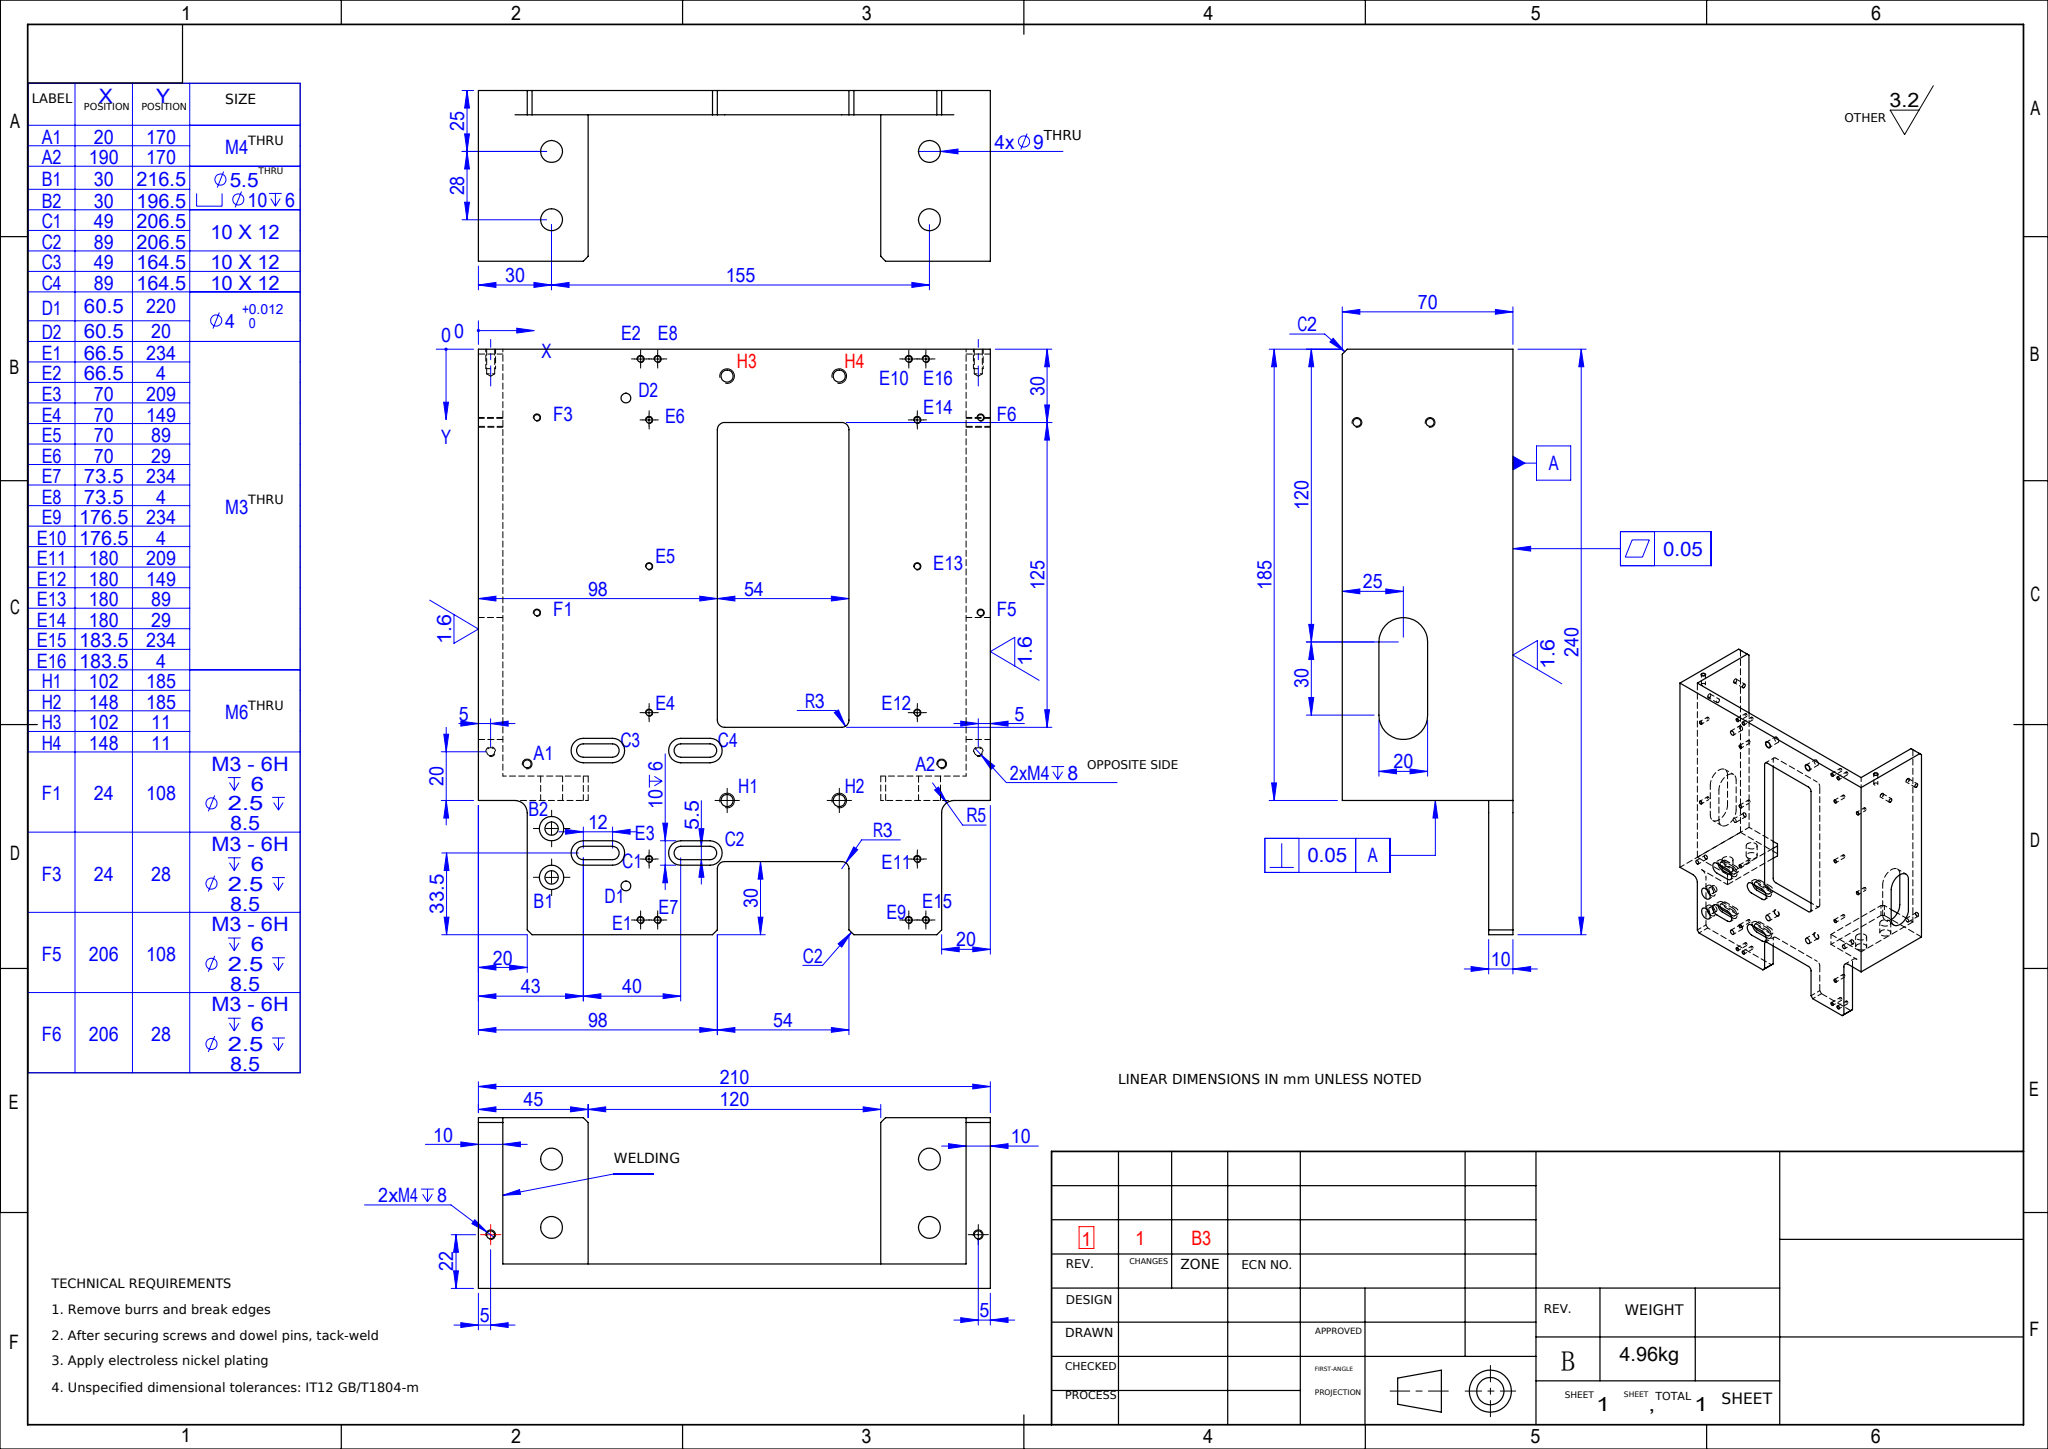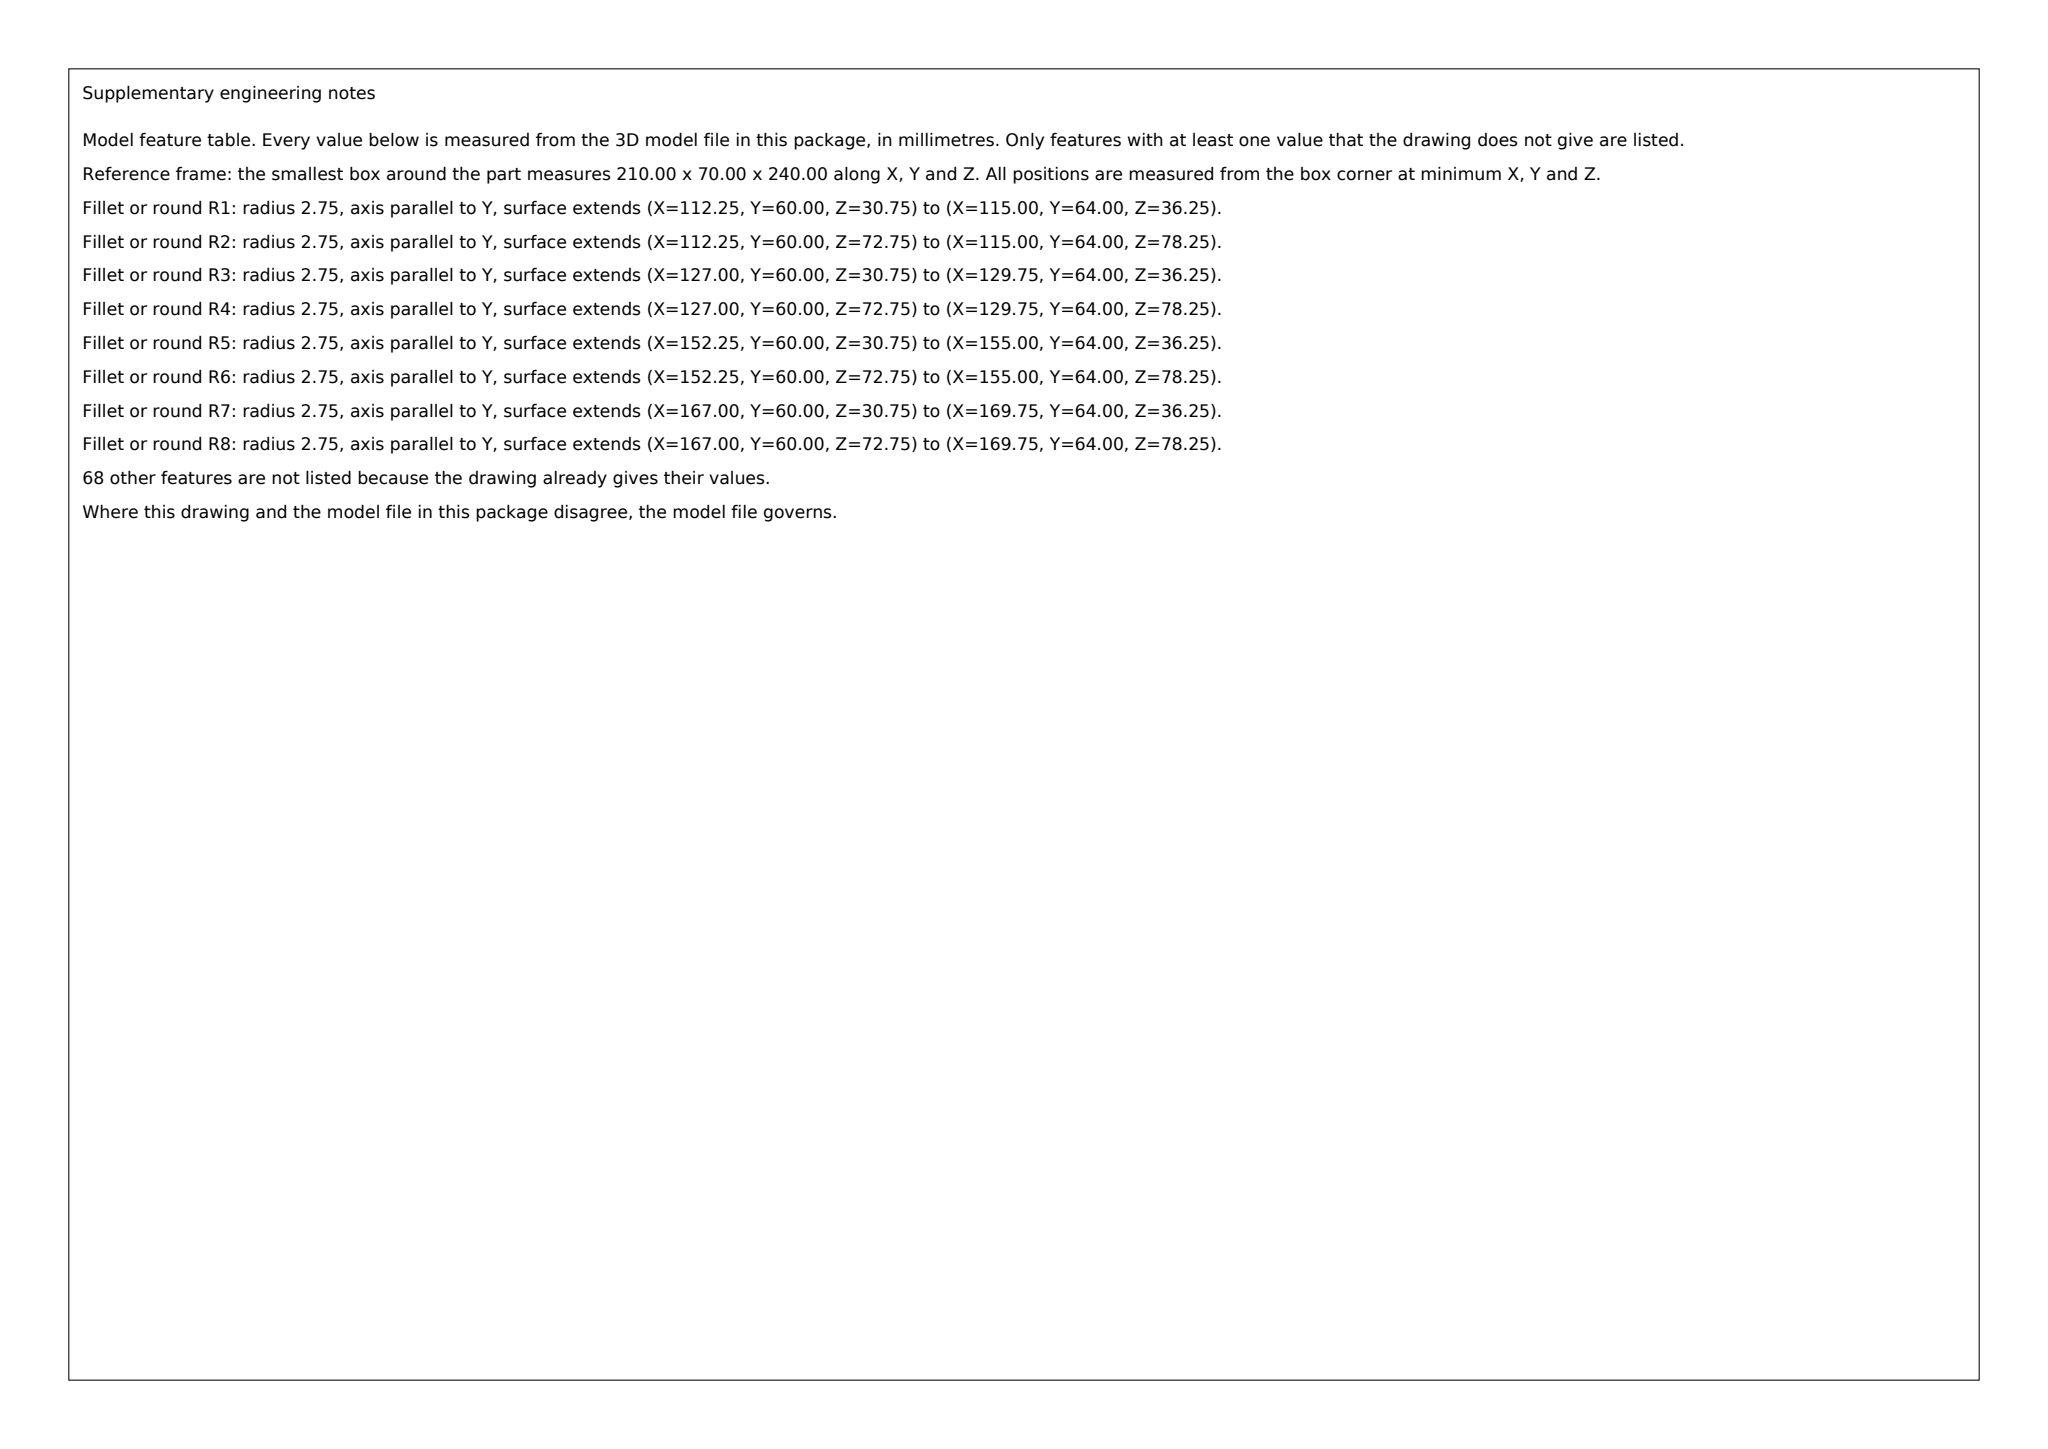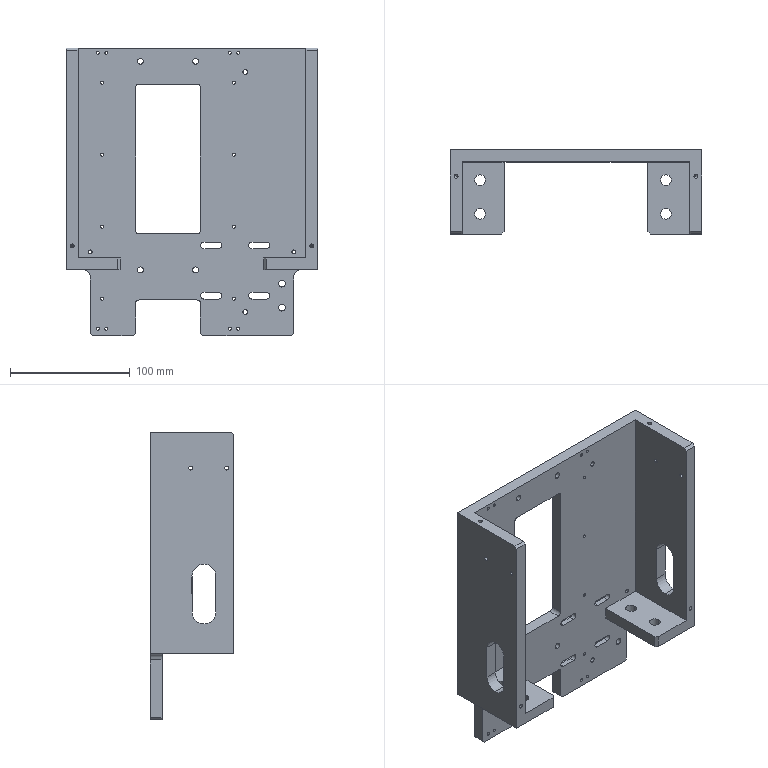Part | SolidWorks | mm | 1 solid | 194 faces | box 210 x 70 x 240 mm | volume 631314 mm3 | cylinder 118 | plane 60 | cone 16 | commonest cylinder face diameters 2.5 x40 3.3 x20 10 x14 5.5 x12 9 x8 5 x8 20 x6 6 x6